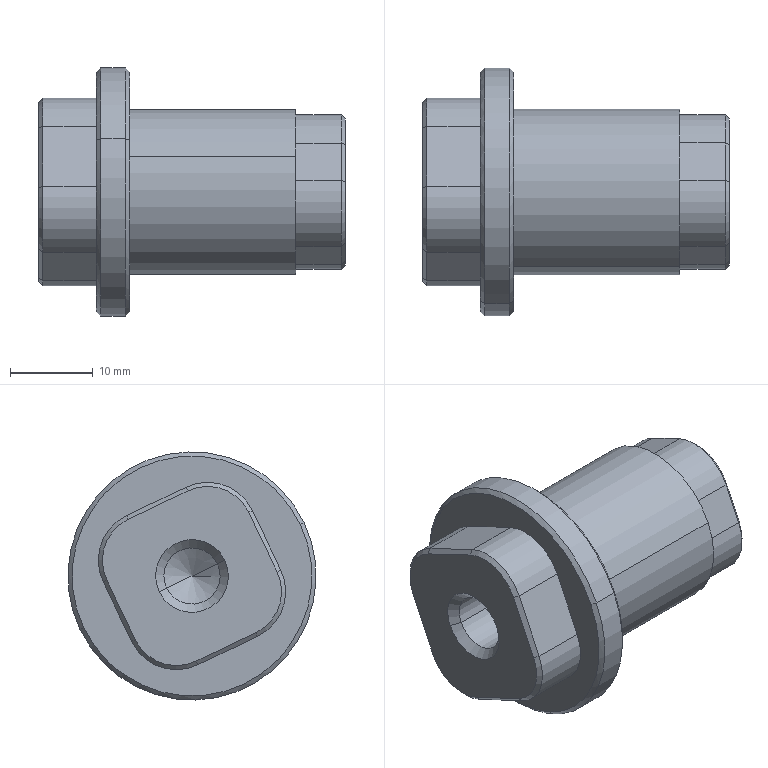Component | SolidWorks | RotationAxis-1 | 1 solid | 57 faces | volume 12400 mm3 | plane 21 | cone 20 | cylinder 16 | commonest cylinder face diameters 12 x8 5 x2 6.8 x2 20 x2 30 x2